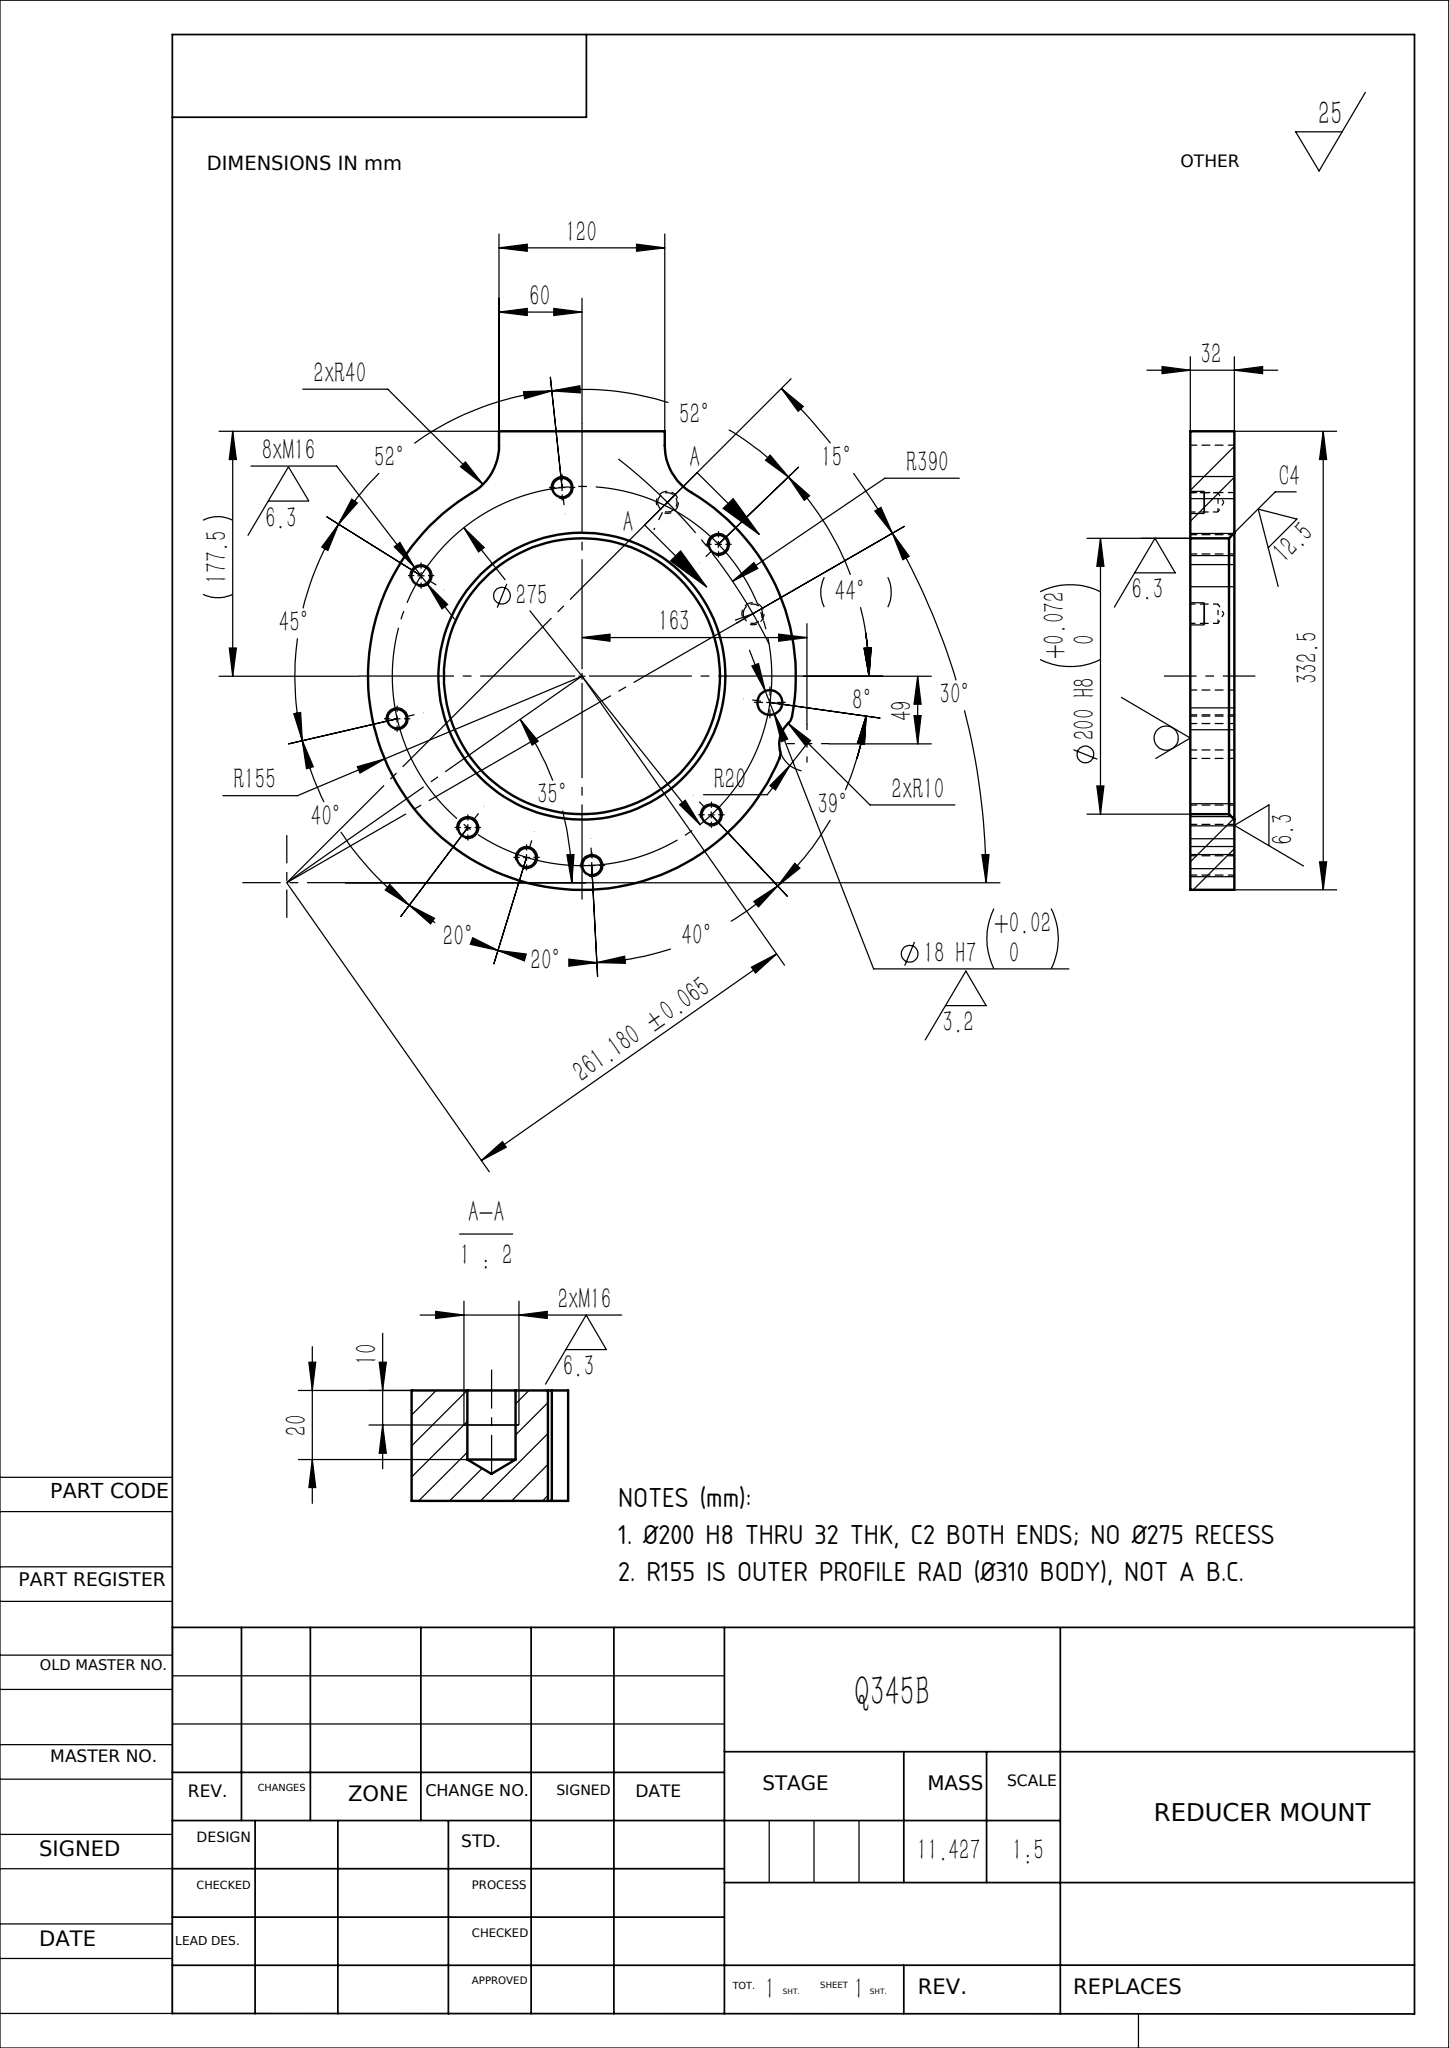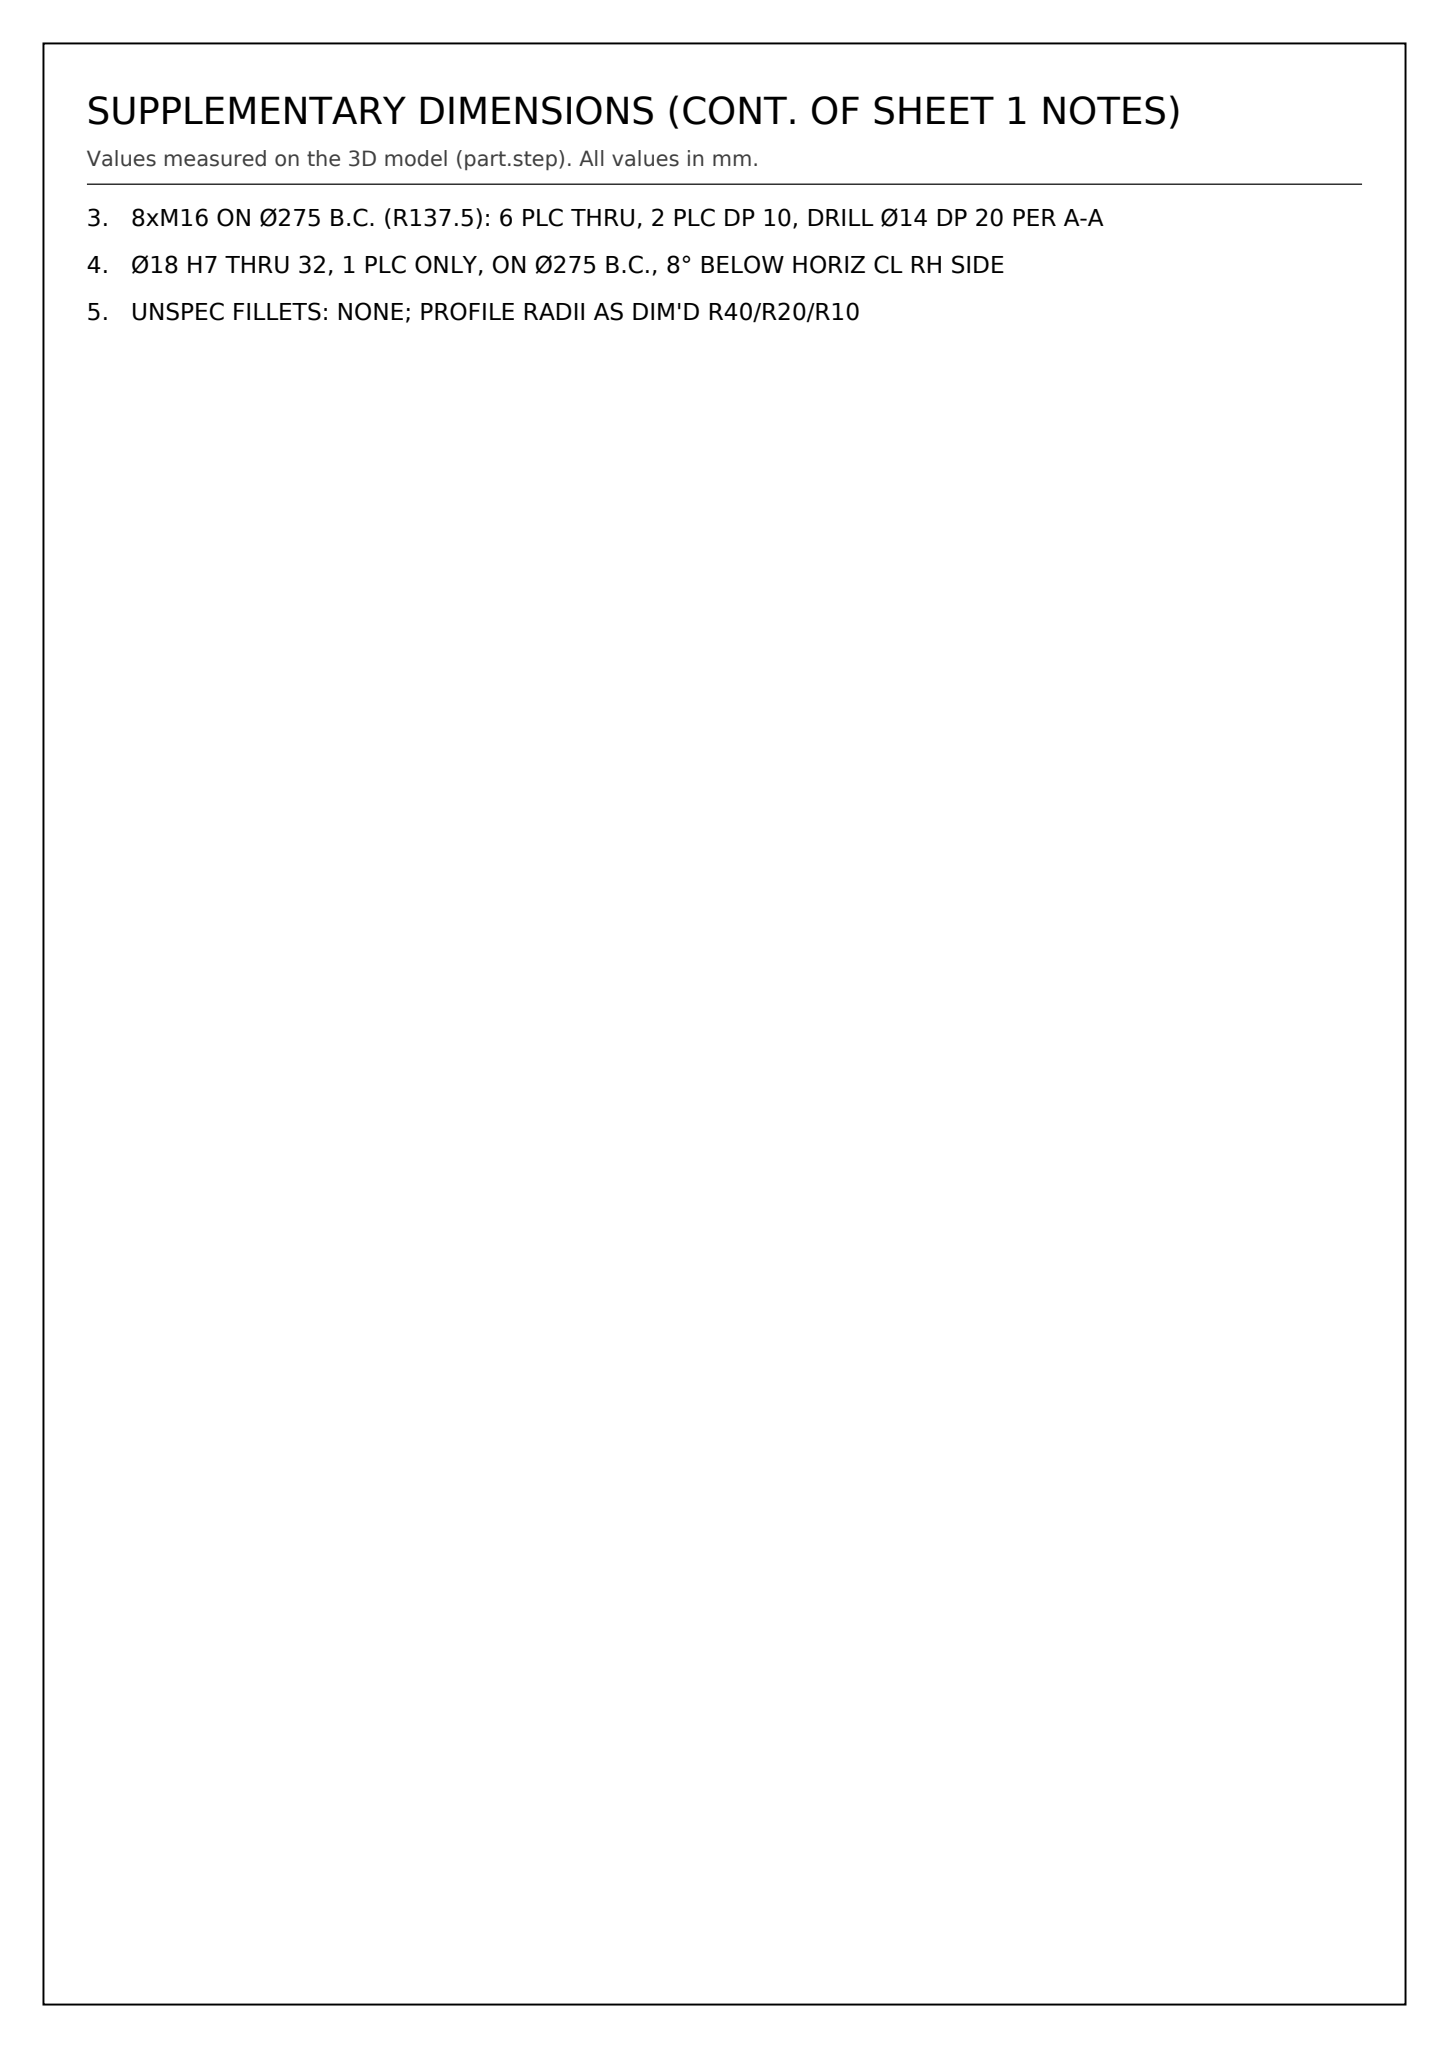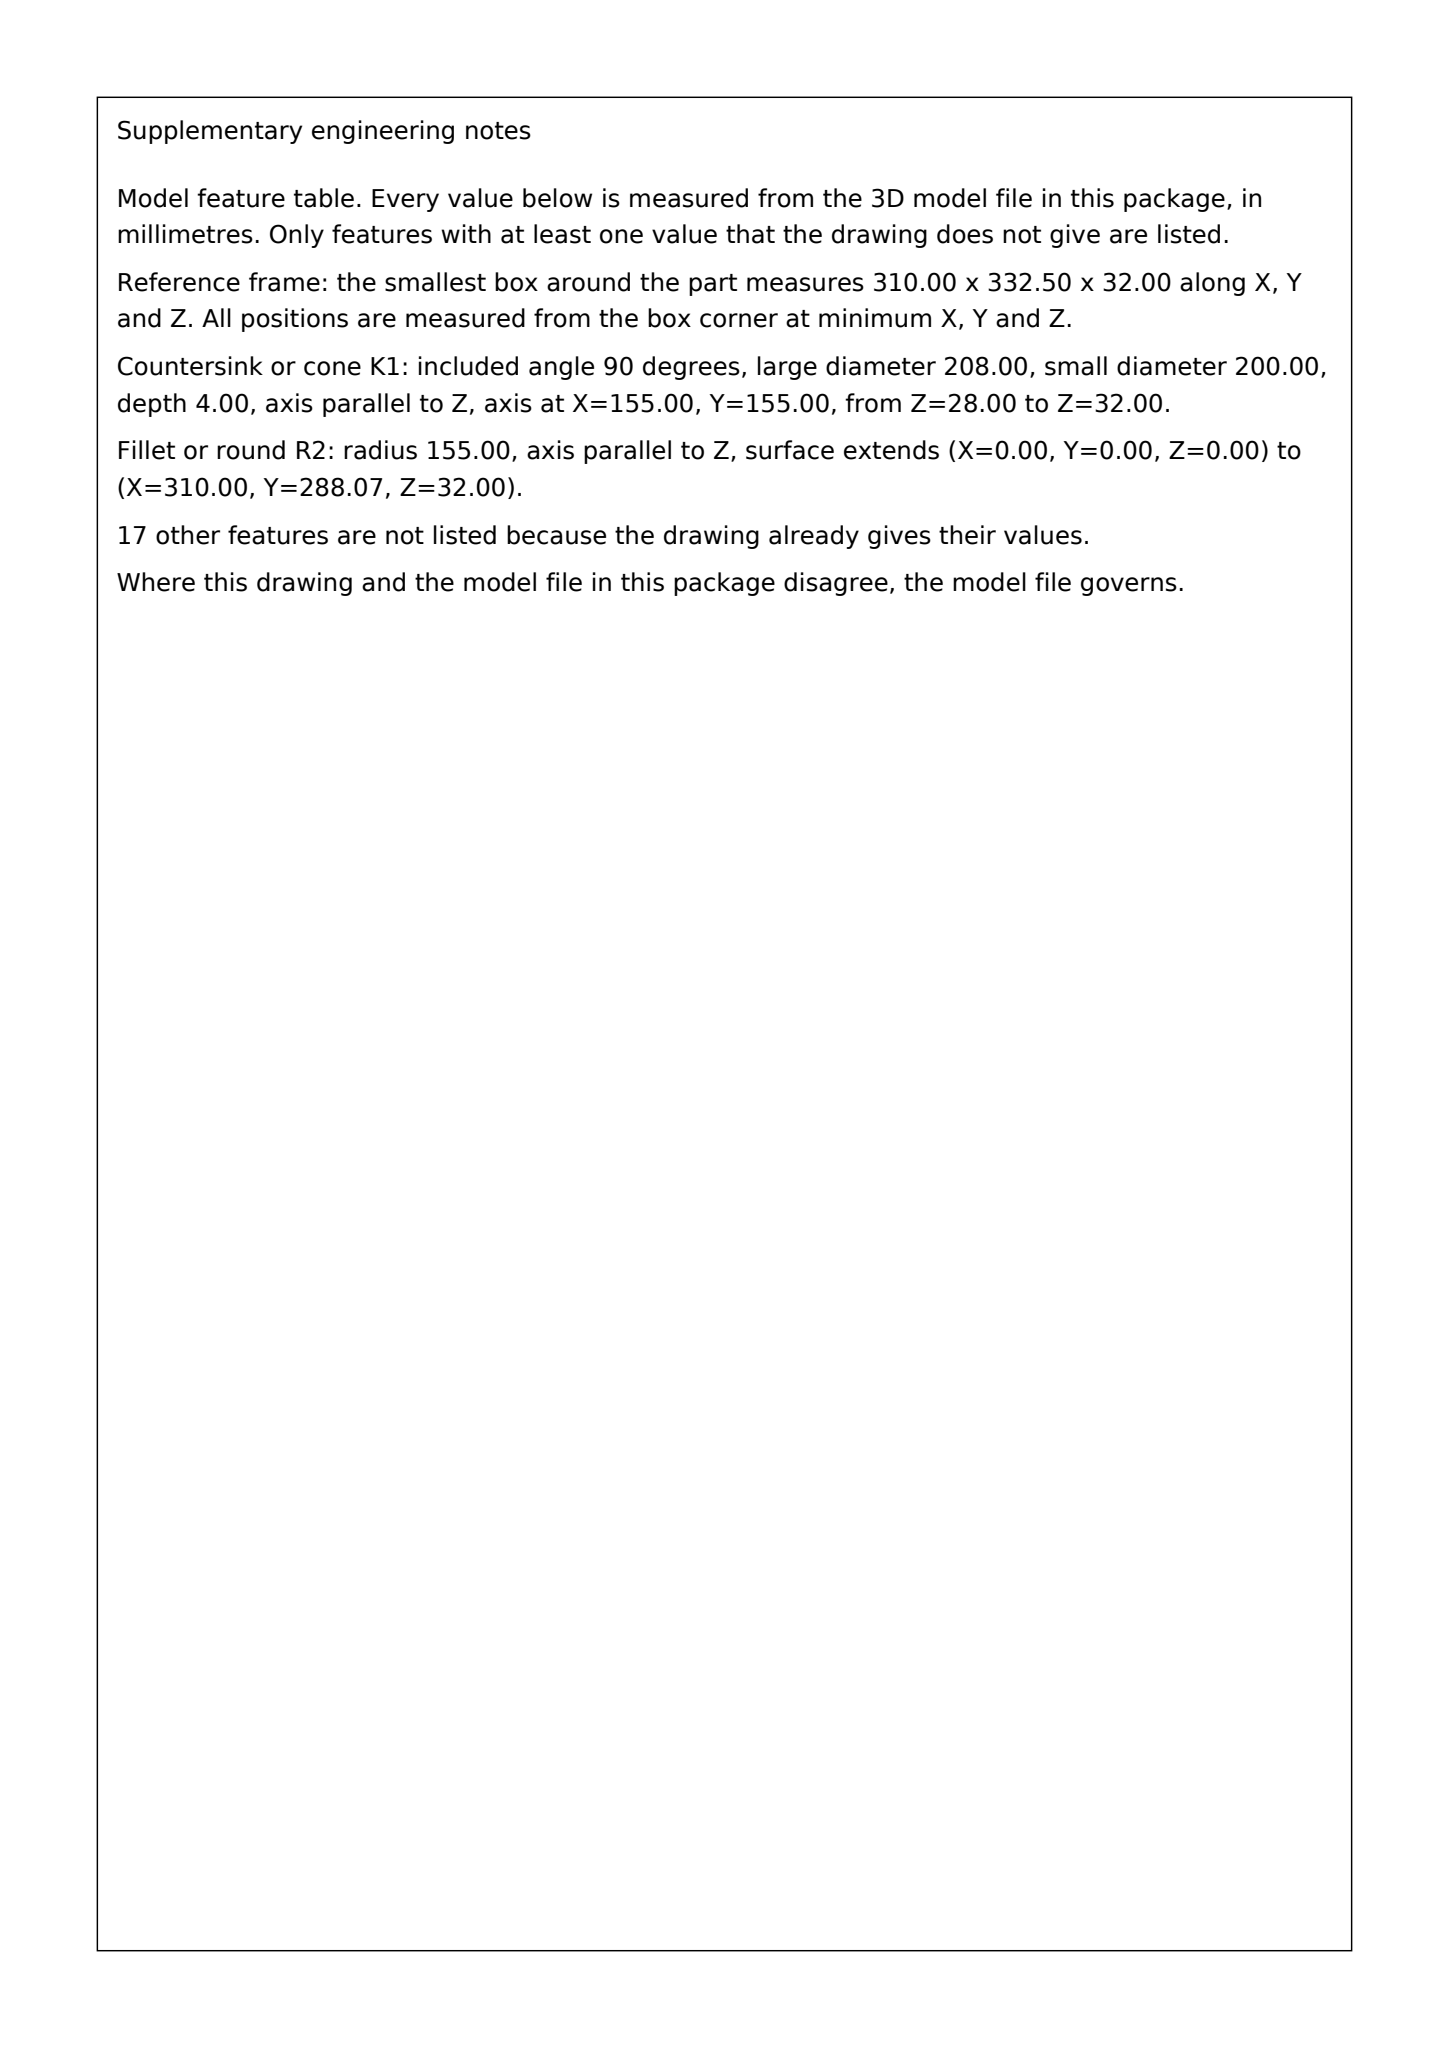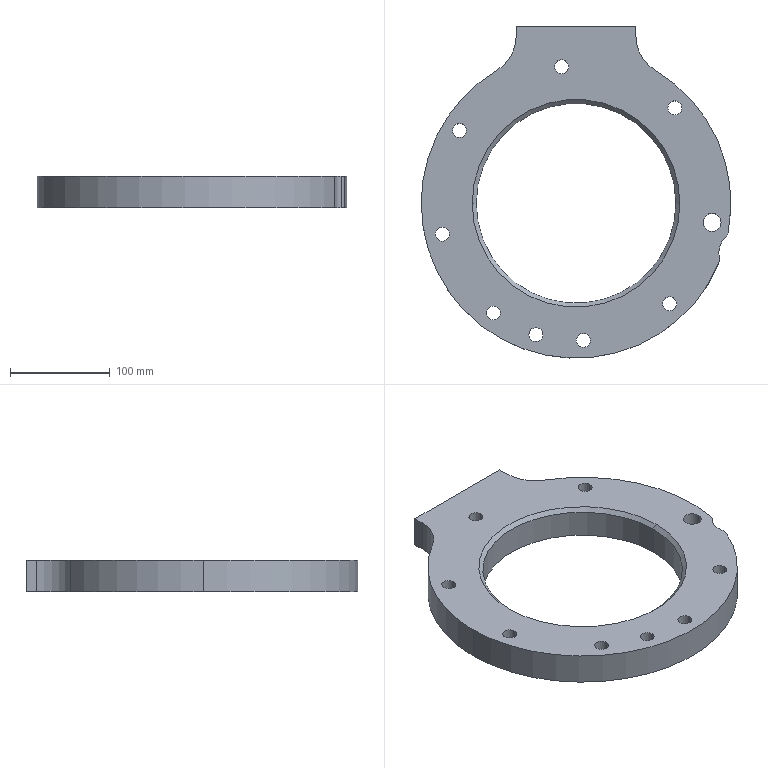Part | SolidWorks | mm | 1 solid | 44 faces | box 310 x 332.5 x 32 mm | volume 1455675 mm3 | cylinder 33 | cone 6 | plane 5 | commonest cylinder face diameters 14 x20 310 x3 18 x2 200 x2 40 x2 80 x2 20 x2
Drawing notes:
Ø200 H8 THRU 32 THK, C2 BOTH ENDS; NO Ø275 RECESS | from the solid: Ø200 cyl L=28 + two 90° cones ref dia 200 (2 deep ea) = 32 total plate thk
R155 IS OUTER PROFILE RAD (Ø310 BODY), NOT A B.C. | from the solid: Outer body cyl Ø310 => R155
8xM16 ON Ø275 B.C. (R137.5): 6 PLC THRU, 2 PLC DP 10, DRILL Ø14 DP 20 PER A-A | from the solid: Eight Ø14 holes at R137.5 from bore axis (155,155); six L=32 thru, two L=20 blind at (216.83,280.96) and (278.80,200.19) with 118° point
Ø18 H7 THRU 32, 1 PLC ONLY, ON Ø275 B.C., 8° BELOW HORIZ CL RH SIDE | from the solid: Single Ø18.0 z-cyl L=32 at (291.16,135.86): R=137.5, angle -8.0° from bore axis
UNSPEC FILLETS: NONE; PROFILE RADII AS DIM'D R40/R20/R10 | from the solid: fillet_radii empty; only Ø80 (R40), Ø40 (R20) and Ø20 (R10) profile arcs exist
build123d program:
from build123d import *

# Parameters (mm, degrees)
SKETCH1_R              = 100
BOSS_EXTRUDE1_DEPTH    = 32
M16_TAPPED_HOLE2_D     = 14
SKETCH5_R              = 9
CUT_EXTRUDE1_DEPTH     = 238.813
CHAMFER1_SIZE          = 4
M16_TAPPED_HOLE3_D     = 14
M16_TAPPED_HOLE3_DEPTH = 20
M16_TAPPED_HOLE3_TIP   = 4.206


with BuildPart() as part:
    # Sketch1 → Boss-Extrude1 (new body)
    with BuildSketch(Plane.XY):
        with BuildLine():
            Line((-60, 167.407), (-60, 177.5))
            Line((-60, 177.5), (60, 177.5))
            Line((60, 177.5), (60, 167.407))
            ThreePointArc((60, 167.407), (65.211, 147.665), (79.487, 133.067))
            ThreePointArc((79.487, 133.067), (141.405, 63.48), (152.257, -29.032))
            ThreePointArc((152.257, -29.032), (151.2, -31.97), (149.289, -34.439))
            ThreePointArc((149.289, -34.439), (143.847, -43.242), (143.533, -53.587))
            ThreePointArc((143.533, -53.587), (143.766, -56.701), (143.027, -59.734))
            ThreePointArc((143.027, -59.734), (-101.501, -117.143), (-79.487, 133.067))
            ThreePointArc((-79.487, 133.067), (-65.211, 147.665), (-60, 167.407))
        make_face()
        Circle(SKETCH1_R, mode=Mode.SUBTRACT)
    extrude(amount=BOSS_EXTRUDE1_DEPTH)

    # M16 Tapped Hole2 (through all)
    with Locations(Plane(origin=(-14.373, 136.747, 32), x_dir=(1, 0, 0), z_dir=(0, 0, 1))):
        with Locations((0, 0), (-102.234, -63.883), (-119.603, -167.678), (-68.377, -246.559), (-25.828, -268.239), (21.569, -274.058), (108.147, -237.308), (113.282, -41.231)):
            Hole(M16_TAPPED_HOLE2_D / 2)

    # Sketch5 → Cut-Extrude1 (cut, through all)
    with BuildSketch(Plane.XY.offset(32)):
        with Locations((136.162, -19.136)):
            Circle(SKETCH5_R)
    extrude(amount=-CUT_EXTRUDE1_DEPTH, mode=Mode.SUBTRACT)

    # Chamfer1
    chamfer1_edges = [part.edges().sort_by_distance(p)[0] for p in [
        (-100, 0, 32),
    ]]
    chamfer(chamfer1_edges, length=CHAMFER1_SIZE)

    # M16 Tapped Hole3
    with Locations(Plane(origin=(61.826, 125.965, 0), x_dir=(-1, 0, 0), z_dir=(0, 0, -1))):
        with Locations((0, 0), (-61.978, -80.772)):
            Hole(M16_TAPPED_HOLE3_D / 2, depth=M16_TAPPED_HOLE3_DEPTH)
            with Locations((0, 0, -(M16_TAPPED_HOLE3_DEPTH + M16_TAPPED_HOLE3_TIP / 2))):  # 118° drill point
                Cone(0, M16_TAPPED_HOLE3_D / 2, M16_TAPPED_HOLE3_TIP, mode=Mode.SUBTRACT)


solid = part.part